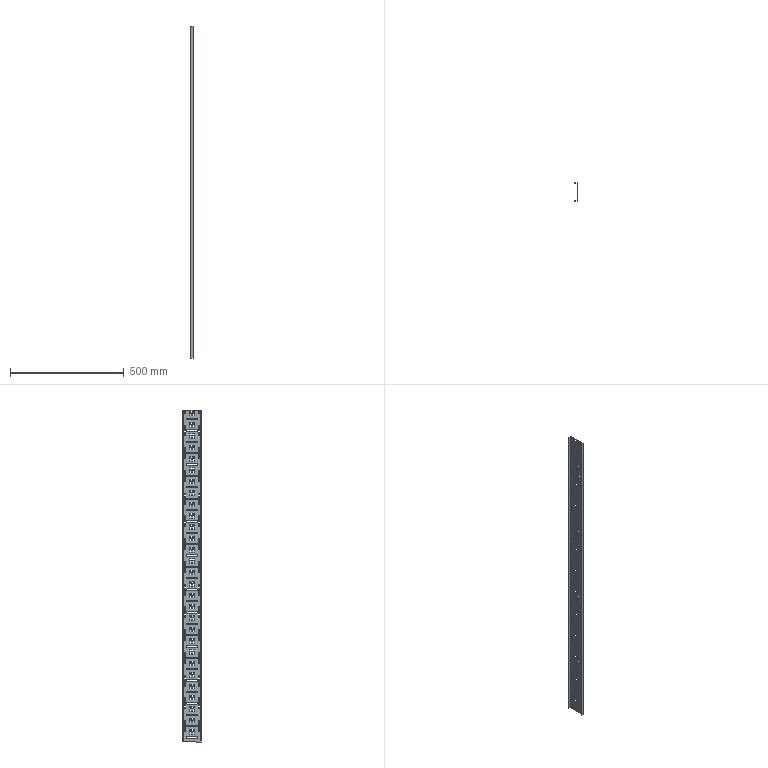Component | SolidWorks | FixedStrip-4 | 1 solid | 636 faces | volume 147060 mm3 | plane 486 | cylinder 150 | commonest cylinder face diameters 6 x146 0.2 x2 2.6 x2